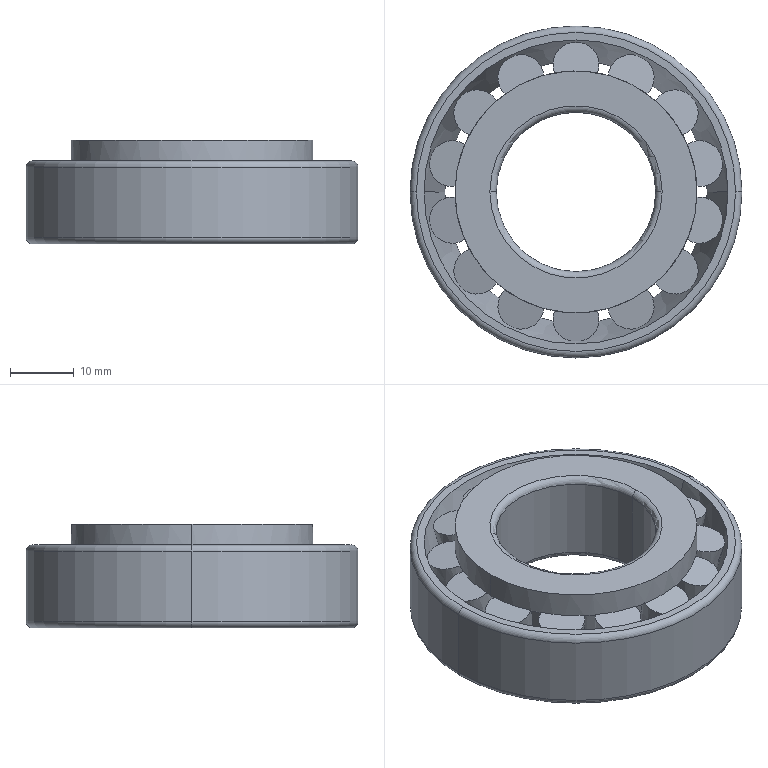Component | SolidWorks | GB_T297-94TaperedRollerBearing30205-2 | 1 solid | 123 faces | volume 18132 mm3 | cone 75 | plane 32 | torus 8 | cylinder 8 | commonest cylinder face diameters 52 x2 25 x2 34.681 x2 37.908 x2